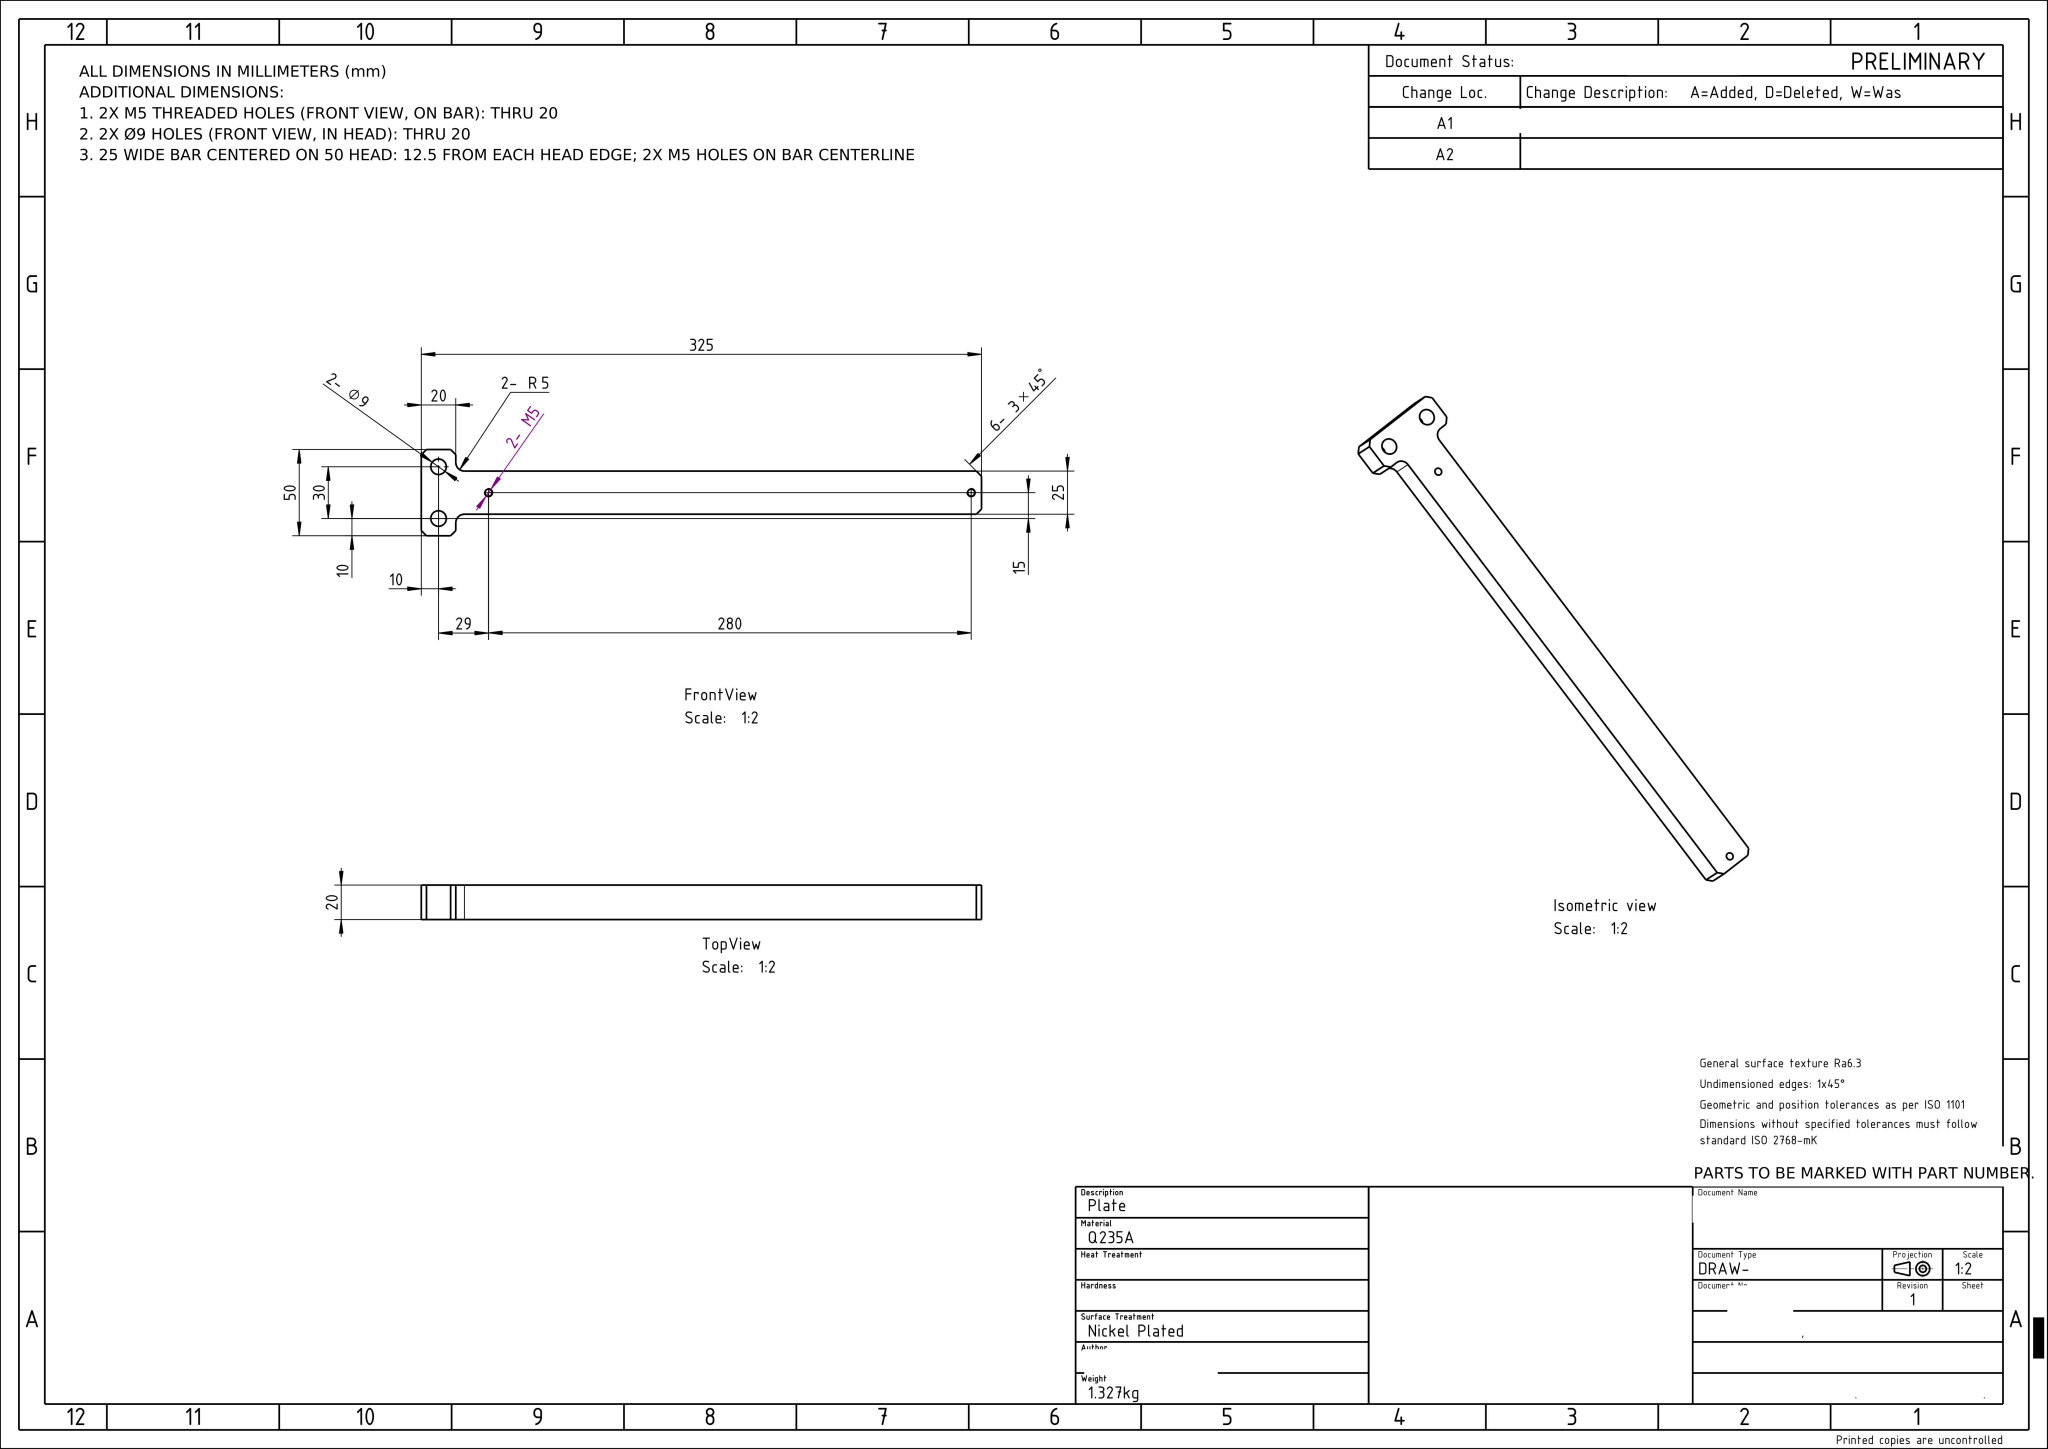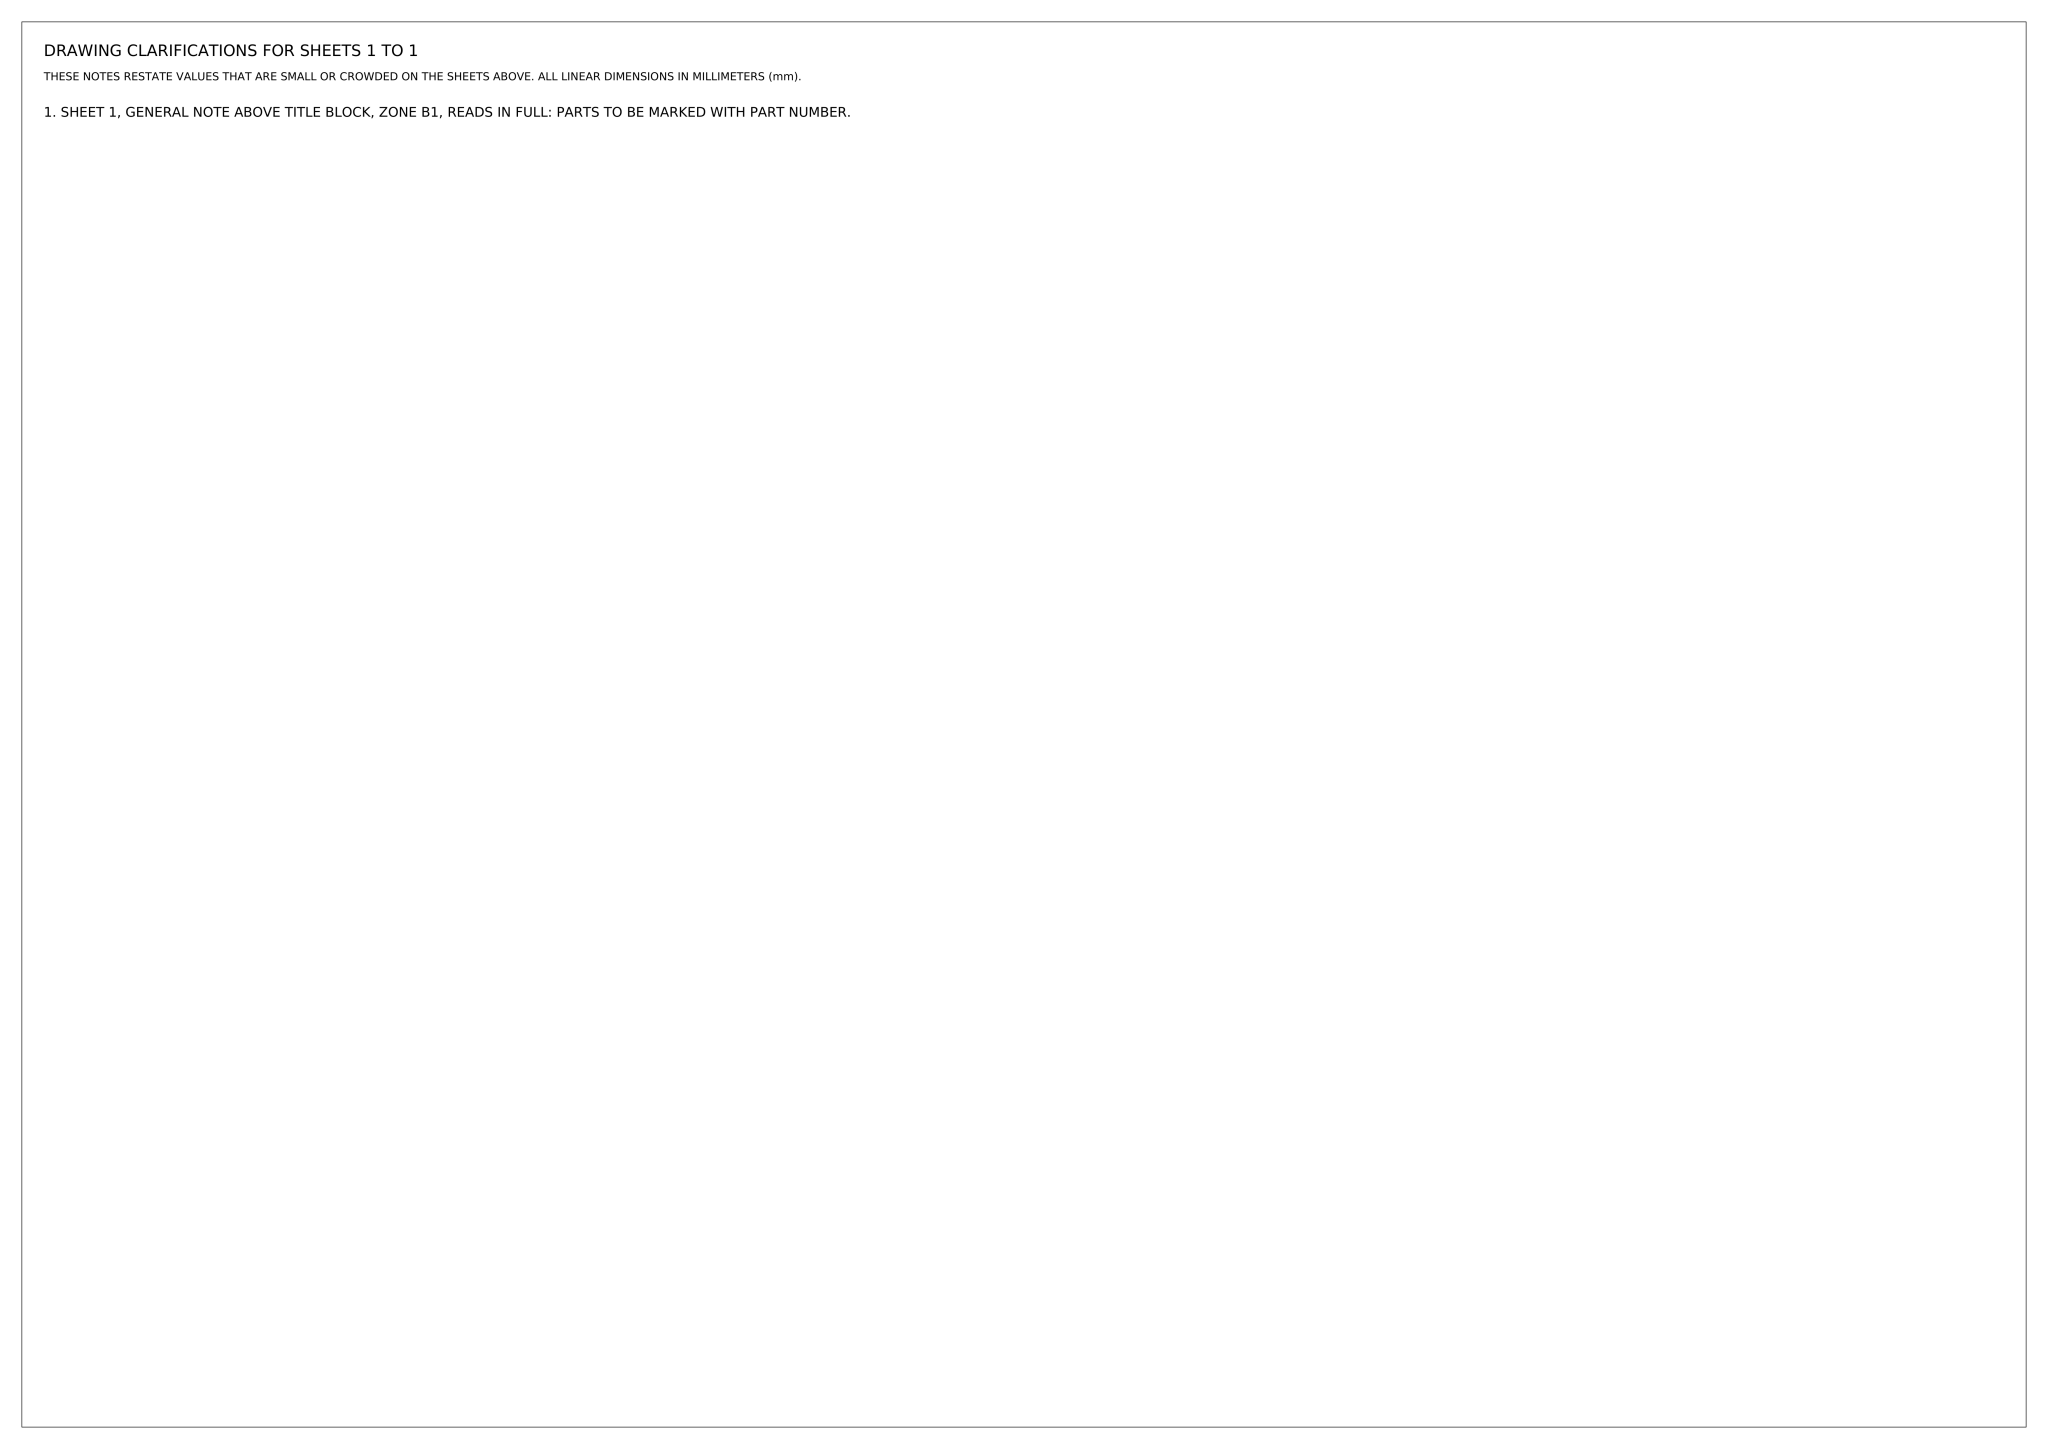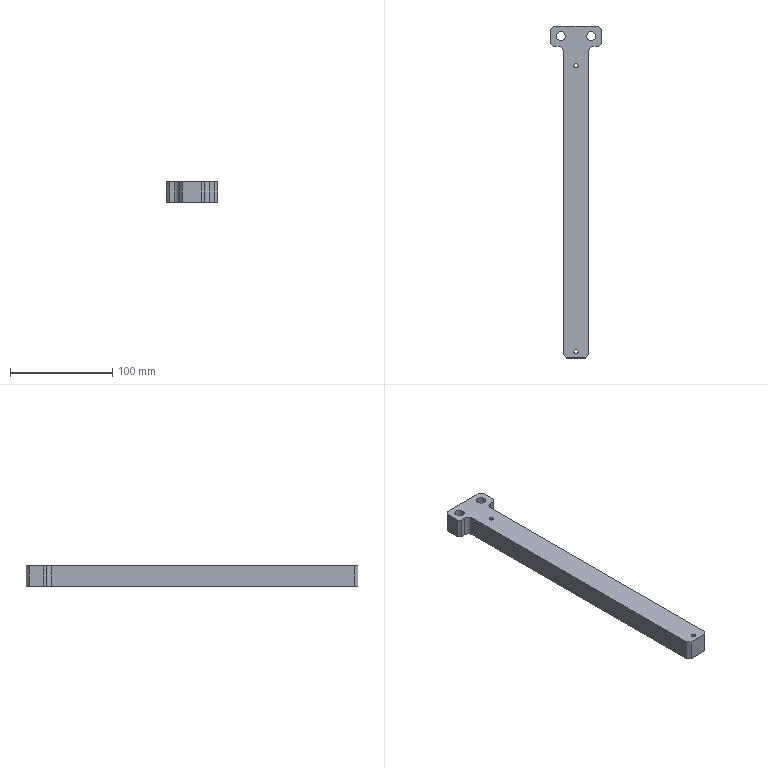Part | NX | mm | 1 solid | 22 faces | box 50 x 325 x 20 mm | volume 169076 mm3 | plane 16 | cylinder 6 | commonest cylinder face diameters 9 x2 4.2 x2 10 x2